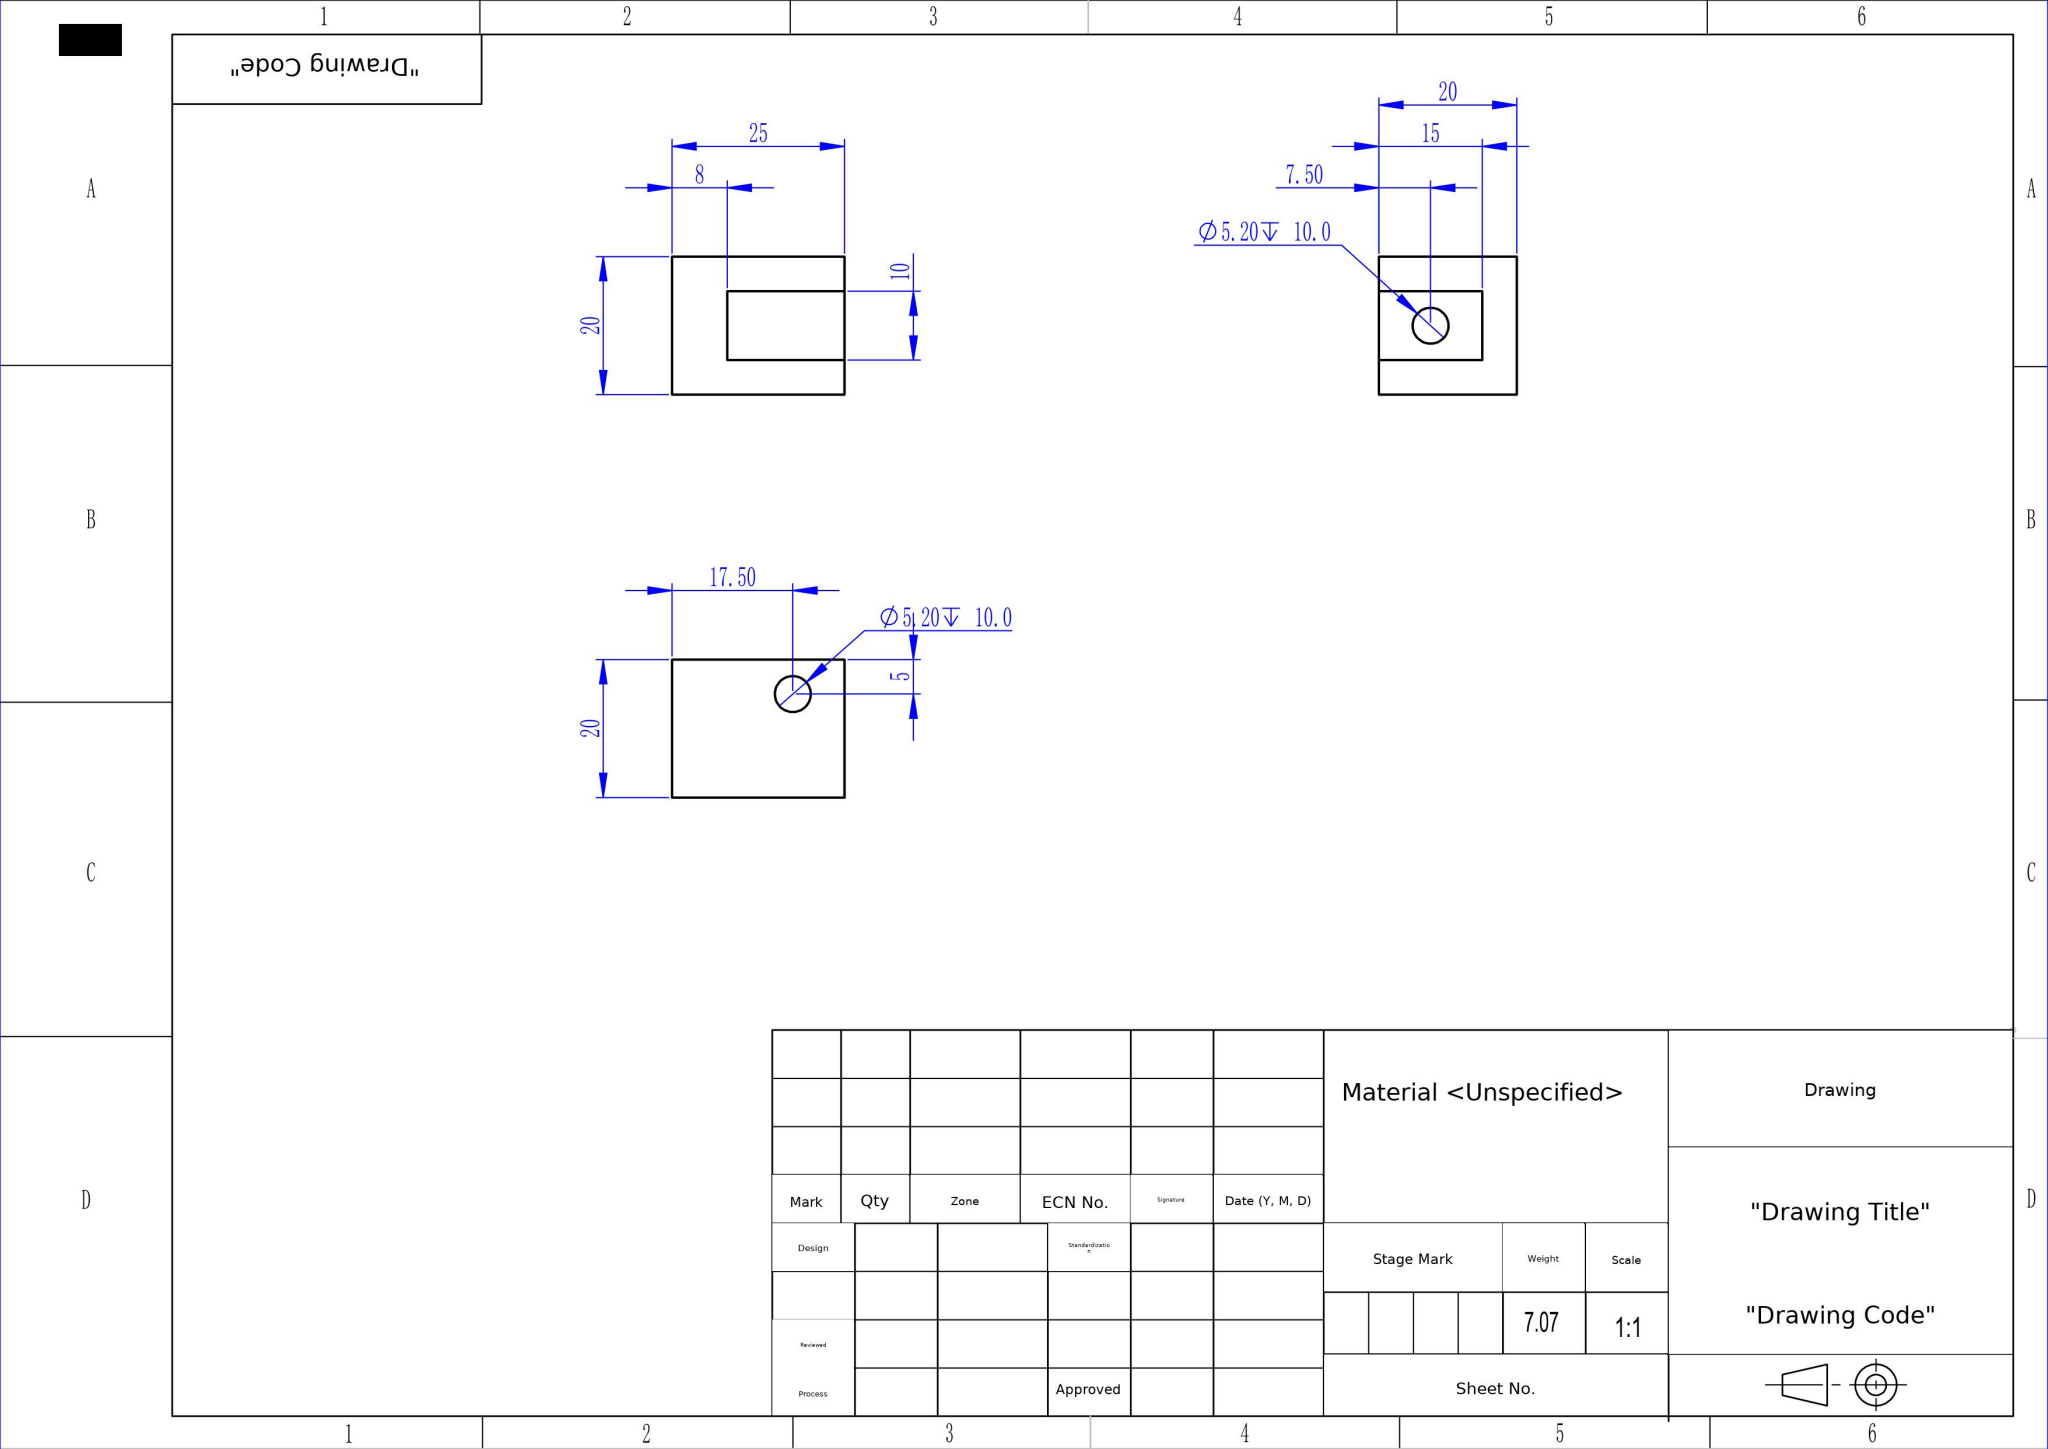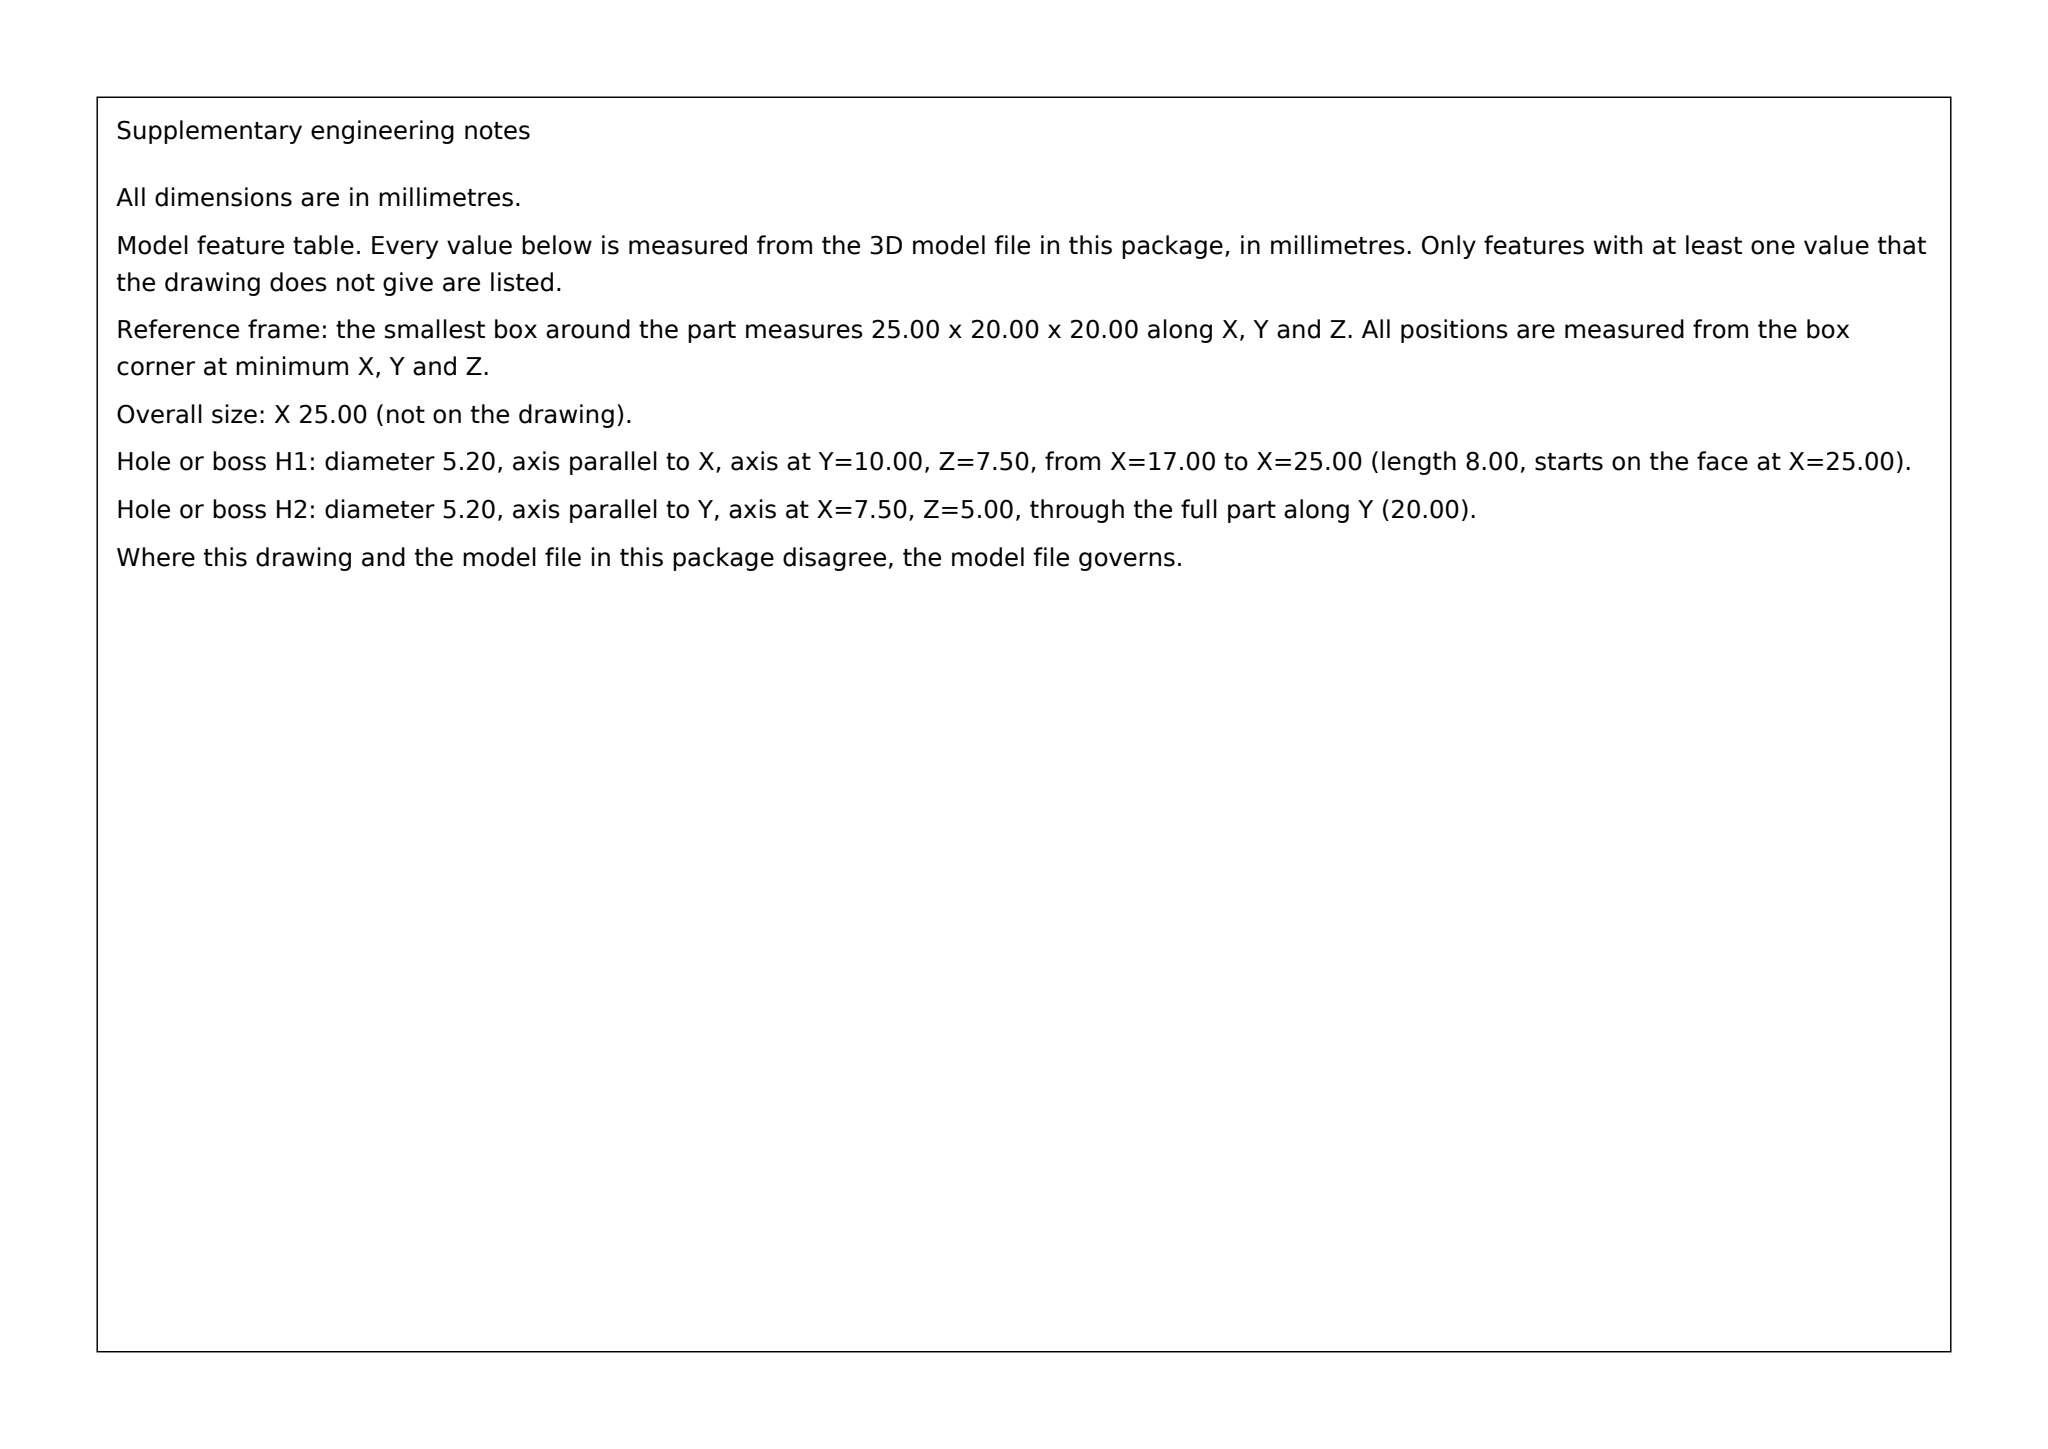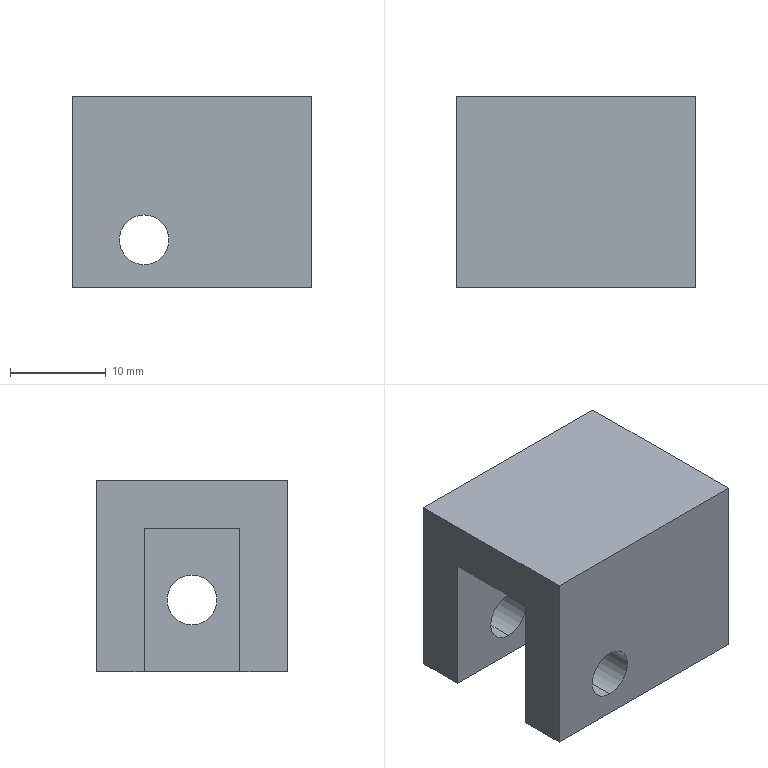Part | SolidWorks | mm | 1 solid | 16 faces | box 25 x 20 x 20 mm | volume 7068 mm3 | plane 10 | cylinder 6 | commonest cylinder face diameters 5.2 x6
build123d program:
from build123d import *

# Parameters (mm, degrees)
SKETCH1_W               = 20
SKETCH1_H               = 20
BOSS_EXTRUDE1_DEPTH     = 25
SKETCH2_W               = 17
SKETCH2_H               = 5
CUT_EXTRUDE1_DEPTH      = 15
SKETCH3_R               = 2.6
CUT_EXTRUDE2_DEPTH      = 10
CUT_EXTRUDE3_DEPTH      = 15
CUT_EXTRUDE3_DEPTH_BACK = 10
SKETCH5_R               = 2.6


with BuildPart() as part:
    # Sketch1 → Boss-Extrude1 (new body)
    with BuildSketch(Plane(origin=(0, 0, 0), x_dir=(0, 0, -1), z_dir=(1, 0, 0))):
        Rectangle(SKETCH1_W, SKETCH1_H)
    extrude(amount=BOSS_EXTRUDE1_DEPTH)

    # Sketch2 → Cut-Extrude1 (cut)
    with BuildSketch(Plane(origin=(0, 0, -10), x_dir=(-1, 0, 0), z_dir=(0, 0, -1))):
        with Locations((-8.5, 2.5)):
            Rectangle(SKETCH2_W, SKETCH2_H)
        with Locations((-8.5, -2.5)):
            Rectangle(SKETCH2_W, SKETCH2_H)
    extrude(amount=-CUT_EXTRUDE1_DEPTH, mode=Mode.SUBTRACT)

    # Sketch3 → Cut-Extrude2 (cut)
    with BuildSketch(Plane.ZY.offset(-17)):
        with Locations((-2.5, 0)):
            Circle(SKETCH3_R)
    extrude(amount=-CUT_EXTRUDE2_DEPTH, mode=Mode.SUBTRACT)

    # Sketch5 → Cut-Extrude3 (cut, two sides: drawn at the far end of the back side and taken through both)
    with BuildSketch(Plane(origin=(0, -5, 0), x_dir=(1, 0, 0), z_dir=(0, 1, 0)).offset(-CUT_EXTRUDE3_DEPTH_BACK)):
        with Locations(Location((7.5, 5, 0), (0, 0, 270))):
            Circle(SKETCH5_R)
    extrude(amount=CUT_EXTRUDE3_DEPTH + CUT_EXTRUDE3_DEPTH_BACK, mode=Mode.SUBTRACT)


solid = part.part
STEP:
#1=CARTESIAN_POINT('',(7.5,10.,-7.6));
#2=VERTEX_POINT('',#1);
#3=CARTESIAN_POINT('',(7.5,10.,-2.4));
#4=VERTEX_POINT('',#3);
#5=CARTESIAN_POINT('',(7.5,10.,-5.));
#6=DIRECTION('',(0.,1.,0.));
#7=DIRECTION('',(0.,0.,1.));
#8=AXIS2_PLACEMENT_3D('',#5,#6,#7);
#9=CIRCLE('',#8,2.6);
#10=EDGE_CURVE('',#2,#4,#9,.T.);
#11=ORIENTED_EDGE('',*,*,#10,.T.);
#12=CARTESIAN_POINT('',(7.5,5.,-2.4));
#13=VERTEX_POINT('',#12);
#14=CARTESIAN_POINT('',(7.5,10.,-2.4));
#15=DIRECTION('',(0.,-1.,-0.));
#16=VECTOR('',#15,1000.);
#17=LINE('',#14,#16);
#18=EDGE_CURVE('',#4,#13,#17,.T.);
#19=ORIENTED_EDGE('',*,*,#18,.T.);
#20=CARTESIAN_POINT('',(7.5,5.,-7.6));
#21=VERTEX_POINT('',#20);
#22=CARTESIAN_POINT('',(7.5,5.,-5.));
#23=DIRECTION('',(-0.,-1.,-0.));
#24=DIRECTION('',(0.,-0.,1.));
#25=AXIS2_PLACEMENT_3D('',#22,#23,#24);
#26=CIRCLE('',#25,2.6);
#27=EDGE_CURVE('',#13,#21,#26,.T.);
#28=ORIENTED_EDGE('',*,*,#27,.T.);
#29=CARTESIAN_POINT('',(7.5,10.,-7.6));
#30=DIRECTION('',(0.,-1.,-0.));
#31=VECTOR('',#30,1000.);
#32=LINE('',#29,#31);
#33=EDGE_CURVE('',#2,#21,#32,.T.);
#34=ORIENTED_EDGE('',*,*,#33,.F.);
#35=EDGE_LOOP('',(#11,#19,#28,#34));
#36=FACE_OUTER_BOUND('',#35,.T.);
#37=CARTESIAN_POINT('',(7.5,10.,-5.));
#38=DIRECTION('',(0.,-1.,-0.));
#39=DIRECTION('',(0.,0.,-1.));
#40=AXIS2_PLACEMENT_3D('',#37,#38,#39);
#41=CYLINDRICAL_SURFACE('',#40,2.6);
#42=ADVANCED_FACE('',(#36),#41,.F.);
#43=CARTESIAN_POINT('',(7.5,-5.,-2.4));
#44=VERTEX_POINT('',#43);
#45=CARTESIAN_POINT('',(7.5,-5.,-7.6));
#46=VERTEX_POINT('',#45);
#47=CARTESIAN_POINT('',(7.5,-5.,-5.));
#48=DIRECTION('',(-0.,-1.,-0.));
#49=DIRECTION('',(0.,-0.,1.));
#50=AXIS2_PLACEMENT_3D('',#47,#48,#49);
#51=CIRCLE('',#50,2.6);
#52=EDGE_CURVE('',#44,#46,#51,.T.);
#53=ORIENTED_EDGE('',*,*,#52,.F.);
#54=CARTESIAN_POINT('',(7.5,-10.,-2.4));
#55=VERTEX_POINT('',#54);
#56=CARTESIAN_POINT('',(7.5,10.,-2.4));
#57=DIRECTION('',(0.,-1.,-0.));
#58=VECTOR('',#57,1000.);
#59=LINE('',#56,#58);
#60=EDGE_CURVE('',#44,#55,#59,.T.);
#61=ORIENTED_EDGE('',*,*,#60,.T.);
#62=CARTESIAN_POINT('',(7.5,-10.,-7.6));
#63=VERTEX_POINT('',#62);
#64=CARTESIAN_POINT('',(7.5,-10.,-5.));
#65=DIRECTION('',(0.,-1.,0.));
#66=DIRECTION('',(0.,0.,1.));
#67=AXIS2_PLACEMENT_3D('',#64,#65,#66);
#68=CIRCLE('',#67,2.6);
#69=EDGE_CURVE('',#55,#63,#68,.T.);
#70=ORIENTED_EDGE('',*,*,#69,.T.);
#71=CARTESIAN_POINT('',(7.5,10.,-7.6));
#72=DIRECTION('',(0.,-1.,-0.));
#73=VECTOR('',#72,1000.);
#74=LINE('',#71,#73);
#75=EDGE_CURVE('',#46,#63,#74,.T.);
#76=ORIENTED_EDGE('',*,*,#75,.F.);
#77=EDGE_LOOP('',(#53,#61,#70,#76));
#78=FACE_OUTER_BOUND('',#77,.T.);
#79=CARTESIAN_POINT('',(7.5,10.,-5.));
#80=DIRECTION('',(0.,-1.,-0.));
#81=DIRECTION('',(0.,0.,-1.));
#82=AXIS2_PLACEMENT_3D('',#79,#80,#81);
#83=CYLINDRICAL_SURFACE('',#82,2.6);
#84=ADVANCED_FACE('',(#78),#83,.F.);
#85=CARTESIAN_POINT('',(25.,0.,0.1));
#86=VERTEX_POINT('',#85);
#87=CARTESIAN_POINT('',(25.,0.,-5.1));
#88=VERTEX_POINT('',#87);
#89=CARTESIAN_POINT('',(25.,0.,-2.5));
#90=DIRECTION('',(1.,0.,0.));
#91=DIRECTION('',(0.,0.,-1.));
#92=AXIS2_PLACEMENT_3D('',#89,#90,#91);
#93=CIRCLE('',#92,2.6);
#94=EDGE_CURVE('',#86,#88,#93,.T.);
#95=ORIENTED_EDGE('',*,*,#94,.T.);
#96=CARTESIAN_POINT('',(17.,0.,-5.1));
#97=VERTEX_POINT('',#96);
#98=CARTESIAN_POINT('',(27.,0.,-5.1));
#99=DIRECTION('',(-1.,0.,0.));
#100=VECTOR('',#99,1000.);
#101=LINE('',#98,#100);
#102=EDGE_CURVE('',#88,#97,#101,.T.);
#103=ORIENTED_EDGE('',*,*,#102,.T.);
#104=CARTESIAN_POINT('',(17.,0.,0.1));
#105=VERTEX_POINT('',#104);
#106=CARTESIAN_POINT('',(17.,0.,-2.5));
#107=DIRECTION('',(-1.,0.,0.));
#108=DIRECTION('',(0.,0.,1.));
#109=AXIS2_PLACEMENT_3D('',#106,#107,#108);
#110=CIRCLE('',#109,2.6);
#111=EDGE_CURVE('',#97,#105,#110,.T.);
#112=ORIENTED_EDGE('',*,*,#111,.T.);
#113=CARTESIAN_POINT('',(27.,0.,0.1));
#114=DIRECTION('',(-1.,0.,0.));
#115=VECTOR('',#114,1000.);
#116=LINE('',#113,#115);
#117=EDGE_CURVE('',#86,#105,#116,.T.);
#118=ORIENTED_EDGE('',*,*,#117,.F.);
#119=EDGE_LOOP('',(#95,#103,#112,#118));
#120=FACE_OUTER_BOUND('',#119,.T.);
#121=CARTESIAN_POINT('',(27.,0.,-2.5));
#122=DIRECTION('',(-1.,0.,0.));
#123=DIRECTION('',(0.,0.,1.));
#124=AXIS2_PLACEMENT_3D('',#121,#122,#123);
#125=CYLINDRICAL_SURFACE('',#124,2.6);
#126=ADVANCED_FACE('',(#120),#125,.F.);
#127=CARTESIAN_POINT('',(17.,-5.,-10.));
#128=VERTEX_POINT('',#127);
#129=CARTESIAN_POINT('',(17.,5.,-10.));
#130=VERTEX_POINT('',#129);
#131=CARTESIAN_POINT('',(17.,0.,-10.));
#132=DIRECTION('',(0.,1.,0.));
#133=VECTOR('',#132,1000.);
#134=LINE('',#131,#133);
#135=EDGE_CURVE('',#128,#130,#134,.T.);
#136=ORIENTED_EDGE('',*,*,#135,.T.);
#137=CARTESIAN_POINT('',(0.,5.,-10.));
#138=VERTEX_POINT('',#137);
#139=CARTESIAN_POINT('',(0.,5.,-10.));
#140=DIRECTION('',(1.,-0.,-0.));
#141=VECTOR('',#140,1000.);
#142=LINE('',#139,#141);
#143=EDGE_CURVE('',#138,#130,#142,.T.);
#144=ORIENTED_EDGE('',*,*,#143,.F.);
#145=CARTESIAN_POINT('',(0.,10.,-10.));
#146=VERTEX_POINT('',#145);
#147=CARTESIAN_POINT('',(0.,10.,-10.));
#148=DIRECTION('',(0.,1.,0.));
#149=VECTOR('',#148,1000.);
#150=LINE('',#147,#149);
#151=EDGE_CURVE('',#138,#146,#150,.T.);
#152=ORIENTED_EDGE('',*,*,#151,.T.);
#153=CARTESIAN_POINT('',(25.,10.,-10.));
#154=VERTEX_POINT('',#153);
#155=CARTESIAN_POINT('',(25.,10.,-10.));
#156=DIRECTION('',(-1.,0.,0.));
#157=VECTOR('',#156,1000.);
#158=LINE('',#155,#157);
#159=EDGE_CURVE('',#154,#146,#158,.T.);
#160=ORIENTED_EDGE('',*,*,#159,.F.);
#161=CARTESIAN_POINT('',(25.,-10.,-10.));
#162=VERTEX_POINT('',#161);
#163=CARTESIAN_POINT('',(25.,10.,-10.));
#164=DIRECTION('',(0.,1.,0.));
#165=VECTOR('',#164,1000.);
#166=LINE('',#163,#165);
#167=EDGE_CURVE('',#162,#154,#166,.T.);
#168=ORIENTED_EDGE('',*,*,#167,.F.);
#169=CARTESIAN_POINT('',(0.,-10.,-10.));
#170=VERTEX_POINT('',#169);
#171=CARTESIAN_POINT('',(25.,-10.,-10.));
#172=DIRECTION('',(-1.,0.,0.));
#173=VECTOR('',#172,1000.);
#174=LINE('',#171,#173);
#175=EDGE_CURVE('',#162,#170,#174,.T.);
#176=ORIENTED_EDGE('',*,*,#175,.T.);
#177=CARTESIAN_POINT('',(0.,-5.,-10.));
#178=VERTEX_POINT('',#177);
#179=CARTESIAN_POINT('',(0.,10.,-10.));
#180=DIRECTION('',(0.,1.,0.));
#181=VECTOR('',#180,1000.);
#182=LINE('',#179,#181);
#183=EDGE_CURVE('',#170,#178,#182,.T.);
#184=ORIENTED_EDGE('',*,*,#183,.T.);
#185=CARTESIAN_POINT('',(-0.,-5.,-10.));
#186=DIRECTION('',(1.,-0.,0.));
#187=VECTOR('',#186,1000.);
#188=LINE('',#185,#187);
#189=EDGE_CURVE('',#178,#128,#188,.T.);
#190=ORIENTED_EDGE('',*,*,#189,.T.);
#191=EDGE_LOOP('',(#136,#144,#152,#160,#168,#176,#184,#190));
#192=FACE_OUTER_BOUND('',#191,.T.);
#193=CARTESIAN_POINT('',(25.,10.,-10.));
#194=DIRECTION('',(0.,-0.,1.));
#195=DIRECTION('',(0.,-1.,-0.));
#196=AXIS2_PLACEMENT_3D('',#193,#194,#195);
#197=PLANE('',#196);
#198=ADVANCED_FACE('',(#192),#197,.F.);
#199=ORIENTED_EDGE('',*,*,#10,.F.);
#200=CARTESIAN_POINT('',(7.5,10.,-5.));
#201=DIRECTION('',(0.,1.,0.));
#202=DIRECTION('',(0.,0.,1.));
#203=AXIS2_PLACEMENT_3D('',#200,#201,#202);
#204=CIRCLE('',#203,2.6);
#205=EDGE_CURVE('',#4,#2,#204,.T.);
#206=ORIENTED_EDGE('',*,*,#205,.F.);
#207=EDGE_LOOP('',(#199,#206));
#208=FACE_BOUND('',#207,.T.);
#209=CARTESIAN_POINT('',(0.,10.,10.));
#210=VERTEX_POINT('',#209);
#211=CARTESIAN_POINT('',(0.,10.,10.));
#212=DIRECTION('',(0.,0.,1.));
#213=VECTOR('',#212,1000.);
#214=LINE('',#211,#213);
#215=EDGE_CURVE('',#146,#210,#214,.T.);
#216=ORIENTED_EDGE('',*,*,#215,.T.);
#217=CARTESIAN_POINT('',(25.,10.,10.));
#218=VERTEX_POINT('',#217);
#219=CARTESIAN_POINT('',(25.,10.,10.));
#220=DIRECTION('',(-1.,0.,0.));
#221=VECTOR('',#220,1000.);
#222=LINE('',#219,#221);
#223=EDGE_CURVE('',#218,#210,#222,.T.);
#224=ORIENTED_EDGE('',*,*,#223,.F.);
#225=CARTESIAN_POINT('',(25.,10.,10.));
#226=DIRECTION('',(0.,0.,1.));
#227=VECTOR('',#226,1000.);
#228=LINE('',#225,#227);
#229=EDGE_CURVE('',#154,#218,#228,.T.);
#230=ORIENTED_EDGE('',*,*,#229,.F.);
#231=ORIENTED_EDGE('',*,*,#159,.T.);
#232=EDGE_LOOP('',(#216,#224,#230,#231));
#233=FACE_OUTER_BOUND('',#232,.T.);
#234=CARTESIAN_POINT('',(25.,10.,10.));
#235=DIRECTION('',(0.,-1.,0.));
#236=DIRECTION('',(0.,0.,-1.));
#237=AXIS2_PLACEMENT_3D('',#234,#235,#236);
#238=PLANE('',#237);
#239=ADVANCED_FACE('',(#208,#233),#238,.F.);
#240=CARTESIAN_POINT('',(0.,-10.,10.));
#241=VERTEX_POINT('',#240);
#242=CARTESIAN_POINT('',(0.,10.,10.));
#243=DIRECTION('',(0.,-1.,-0.));
#244=VECTOR('',#243,1000.);
#245=LINE('',#242,#244);
#246=EDGE_CURVE('',#210,#241,#245,.T.);
#247=ORIENTED_EDGE('',*,*,#246,.T.);
#248=CARTESIAN_POINT('',(25.,-10.,10.));
#249=VERTEX_POINT('',#248);
#250=CARTESIAN_POINT('',(25.,-10.,10.));
#251=DIRECTION('',(-1.,0.,0.));
#252=VECTOR('',#251,1000.);
#253=LINE('',#250,#252);
#254=EDGE_CURVE('',#249,#241,#253,.T.);
#255=ORIENTED_EDGE('',*,*,#254,.F.);
#256=CARTESIAN_POINT('',(25.,10.,10.));
#257=DIRECTION('',(0.,-1.,-0.));
#258=VECTOR('',#257,1000.);
#259=LINE('',#256,#258);
#260=EDGE_CURVE('',#218,#249,#259,.T.);
#261=ORIENTED_EDGE('',*,*,#260,.F.);
#262=ORIENTED_EDGE('',*,*,#223,.T.);
#263=EDGE_LOOP('',(#247,#255,#261,#262));
#264=FACE_OUTER_BOUND('',#263,.T.);
#265=CARTESIAN_POINT('',(25.,10.,10.));
#266=DIRECTION('',(0.,0.,-1.));
#267=DIRECTION('',(0.,1.,0.));
#268=AXIS2_PLACEMENT_3D('',#265,#266,#267);
#269=PLANE('',#268);
#270=ADVANCED_FACE('',(#264),#269,.F.);
#271=CARTESIAN_POINT('',(7.5,-10.,-5.));
#272=DIRECTION('',(0.,-1.,0.));
#273=DIRECTION('',(0.,0.,1.));
#274=AXIS2_PLACEMENT_3D('',#271,#272,#273);
#275=CIRCLE('',#274,2.6);
#276=EDGE_CURVE('',#63,#55,#275,.T.);
#277=ORIENTED_EDGE('',*,*,#276,.F.);
#278=ORIENTED_EDGE('',*,*,#69,.F.);
#279=EDGE_LOOP('',(#277,#278));
#280=FACE_BOUND('',#279,.T.);
#281=CARTESIAN_POINT('',(0.,-10.,10.));
#282=DIRECTION('',(0.,0.,-1.));
#283=VECTOR('',#282,1000.);
#284=LINE('',#281,#283);
#285=EDGE_CURVE('',#241,#170,#284,.T.);
#286=ORIENTED_EDGE('',*,*,#285,.T.);
#287=ORIENTED_EDGE('',*,*,#175,.F.);
#288=CARTESIAN_POINT('',(25.,-10.,10.));
#289=DIRECTION('',(0.,0.,-1.));
#290=VECTOR('',#289,1000.);
#291=LINE('',#288,#290);
#292=EDGE_CURVE('',#249,#162,#291,.T.);
#293=ORIENTED_EDGE('',*,*,#292,.F.);
#294=ORIENTED_EDGE('',*,*,#254,.T.);
#295=EDGE_LOOP('',(#286,#287,#293,#294));
#296=FACE_OUTER_BOUND('',#295,.T.);
#297=CARTESIAN_POINT('',(25.,-10.,10.));
#298=DIRECTION('',(0.,1.,0.));
#299=DIRECTION('',(0.,0.,1.));
#300=AXIS2_PLACEMENT_3D('',#297,#298,#299);
#301=PLANE('',#300);
#302=ADVANCED_FACE('',(#280,#296),#301,.F.);
#303=ORIENTED_EDGE('',*,*,#94,.F.);
#304=CARTESIAN_POINT('',(25.,0.,-2.5));
#305=DIRECTION('',(1.,0.,0.));
#306=DIRECTION('',(0.,0.,-1.));
#307=AXIS2_PLACEMENT_3D('',#304,#305,#306);
#308=CIRCLE('',#307,2.6);
#309=EDGE_CURVE('',#88,#86,#308,.T.);
#310=ORIENTED_EDGE('',*,*,#309,.F.);
#311=EDGE_LOOP('',(#303,#310));
#312=FACE_BOUND('',#311,.T.);
#313=ORIENTED_EDGE('',*,*,#167,.T.);
#314=ORIENTED_EDGE('',*,*,#229,.T.);
#315=ORIENTED_EDGE('',*,*,#260,.T.);
#316=ORIENTED_EDGE('',*,*,#292,.T.);
#317=EDGE_LOOP('',(#313,#314,#315,#316));
#318=FACE_OUTER_BOUND('',#317,.T.);
#319=CARTESIAN_POINT('',(25.,0.,0.));
#320=DIRECTION('',(1.,0.,0.));
#321=DIRECTION('',(0.,0.,-1.));
#322=AXIS2_PLACEMENT_3D('',#319,#320,#321);
#323=PLANE('',#322);
#324=ADVANCED_FACE('',(#312,#318),#323,.T.);
#325=ORIENTED_EDGE('',*,*,#151,.F.);
#326=CARTESIAN_POINT('',(0.,5.,5.));
#327=VERTEX_POINT('',#326);
#328=CARTESIAN_POINT('',(0.,5.,5.));
#329=DIRECTION('',(0.,0.,-1.));
#330=VECTOR('',#329,1000.);
#331=LINE('',#328,#330);
#332=EDGE_CURVE('',#327,#138,#331,.T.);
#333=ORIENTED_EDGE('',*,*,#332,.F.);
#334=CARTESIAN_POINT('',(0.,-5.,5.));
#335=VERTEX_POINT('',#334);
#336=CARTESIAN_POINT('',(0.,-0.,5.));
#337=DIRECTION('',(0.,1.,0.));
#338=VECTOR('',#337,1000.);
#339=LINE('',#336,#338);
#340=EDGE_CURVE('',#335,#327,#339,.T.);
#341=ORIENTED_EDGE('',*,*,#340,.F.);
#342=CARTESIAN_POINT('',(0.,-5.,5.));
#343=DIRECTION('',(0.,0.,-1.));
#344=VECTOR('',#343,1000.);
#345=LINE('',#342,#344);
#346=EDGE_CURVE('',#335,#178,#345,.T.);
#347=ORIENTED_EDGE('',*,*,#346,.T.);
#348=ORIENTED_EDGE('',*,*,#183,.F.);
#349=ORIENTED_EDGE('',*,*,#285,.F.);
#350=ORIENTED_EDGE('',*,*,#246,.F.);
#351=ORIENTED_EDGE('',*,*,#215,.F.);
#352=EDGE_LOOP('',(#325,#333,#341,#347,#348,#349,#350,#351));
#353=FACE_OUTER_BOUND('',#352,.T.);
#354=CARTESIAN_POINT('',(0.,0.,0.));
#355=DIRECTION('',(1.,0.,0.));
#356=DIRECTION('',(0.,0.,-1.));
#357=AXIS2_PLACEMENT_3D('',#354,#355,#356);
#358=PLANE('',#357);
#359=ADVANCED_FACE('',(#353),#358,.F.);
#360=CARTESIAN_POINT('',(17.,0.,-2.5));
#361=DIRECTION('',(-1.,0.,0.));
#362=DIRECTION('',(0.,0.,1.));
#363=AXIS2_PLACEMENT_3D('',#360,#361,#362);
#364=CIRCLE('',#363,2.6);
#365=EDGE_CURVE('',#105,#97,#364,.T.);
#366=ORIENTED_EDGE('',*,*,#365,.F.);
#367=ORIENTED_EDGE('',*,*,#111,.F.);
#368=EDGE_LOOP('',(#366,#367));
#369=FACE_BOUND('',#368,.T.);
#370=ORIENTED_EDGE('',*,*,#135,.F.);
#371=CARTESIAN_POINT('',(17.,-5.,5.));
#372=VERTEX_POINT('',#371);
#373=CARTESIAN_POINT('',(17.,-5.,5.));
#374=DIRECTION('',(0.,0.,-1.));
#375=VECTOR('',#374,1000.);
#376=LINE('',#373,#375);
#377=EDGE_CURVE('',#372,#128,#376,.T.);
#378=ORIENTED_EDGE('',*,*,#377,.F.);
#379=CARTESIAN_POINT('',(17.,5.,5.));
#380=VERTEX_POINT('',#379);
#381=CARTESIAN_POINT('',(17.,-0.,5.));
#382=DIRECTION('',(0.,1.,0.));
#383=VECTOR('',#382,1000.);
#384=LINE('',#381,#383);
#385=EDGE_CURVE('',#372,#380,#384,.T.);
#386=ORIENTED_EDGE('',*,*,#385,.T.);
#387=CARTESIAN_POINT('',(17.,5.,5.));
#388=DIRECTION('',(0.,0.,-1.));
#389=VECTOR('',#388,1000.);
#390=LINE('',#387,#389);
#391=EDGE_CURVE('',#380,#130,#390,.T.);
#392=ORIENTED_EDGE('',*,*,#391,.T.);
#393=EDGE_LOOP('',(#370,#378,#386,#392));
#394=FACE_OUTER_BOUND('',#393,.T.);
#395=CARTESIAN_POINT('',(17.,-0.,5.));
#396=DIRECTION('',(-1.,0.,0.));
#397=DIRECTION('',(0.,0.,1.));
#398=AXIS2_PLACEMENT_3D('',#395,#396,#397);
#399=PLANE('',#398);
#400=ADVANCED_FACE('',(#369,#394),#399,.T.);
#401=CARTESIAN_POINT('',(7.5,5.,-5.));
#402=DIRECTION('',(-0.,-1.,-0.));
#403=DIRECTION('',(0.,-0.,1.));
#404=AXIS2_PLACEMENT_3D('',#401,#402,#403);
#405=CIRCLE('',#404,2.6);
#406=EDGE_CURVE('',#21,#13,#405,.T.);
#407=ORIENTED_EDGE('',*,*,#406,.F.);
#408=ORIENTED_EDGE('',*,*,#27,.F.);
#409=EDGE_LOOP('',(#407,#408));
#410=FACE_BOUND('',#409,.T.);
#411=ORIENTED_EDGE('',*,*,#143,.T.);
#412=ORIENTED_EDGE('',*,*,#391,.F.);
#413=CARTESIAN_POINT('',(0.,5.,5.));
#414=DIRECTION('',(1.,-0.,-0.));
#415=VECTOR('',#414,1000.);
#416=LINE('',#413,#415);
#417=EDGE_CURVE('',#327,#380,#416,.T.);
#418=ORIENTED_EDGE('',*,*,#417,.F.);
#419=ORIENTED_EDGE('',*,*,#332,.T.);
#420=EDGE_LOOP('',(#411,#412,#418,#419));
#421=FACE_OUTER_BOUND('',#420,.T.);
#422=CARTESIAN_POINT('',(0.,5.,5.));
#423=DIRECTION('',(0.,1.,0.));
#424=DIRECTION('',(0.,-0.,1.));
#425=AXIS2_PLACEMENT_3D('',#422,#423,#424);
#426=PLANE('',#425);
#427=ADVANCED_FACE('',(#410,#421),#426,.F.);
#428=CARTESIAN_POINT('',(7.5,-5.,-5.));
#429=DIRECTION('',(-0.,-1.,-0.));
#430=DIRECTION('',(0.,-0.,1.));
#431=AXIS2_PLACEMENT_3D('',#428,#429,#430);
#432=CIRCLE('',#431,2.6);
#433=EDGE_CURVE('',#46,#44,#432,.T.);
#434=ORIENTED_EDGE('',*,*,#433,.T.);
#435=ORIENTED_EDGE('',*,*,#52,.T.);
#436=EDGE_LOOP('',(#434,#435));
#437=FACE_BOUND('',#436,.T.);
#438=ORIENTED_EDGE('',*,*,#189,.F.);
#439=ORIENTED_EDGE('',*,*,#346,.F.);
#440=CARTESIAN_POINT('',(-0.,-5.,5.));
#441=DIRECTION('',(1.,-0.,0.));
#442=VECTOR('',#441,1000.);
#443=LINE('',#440,#442);
#444=EDGE_CURVE('',#335,#372,#443,.T.);
#445=ORIENTED_EDGE('',*,*,#444,.T.);
#446=ORIENTED_EDGE('',*,*,#377,.T.);
#447=EDGE_LOOP('',(#438,#439,#445,#446));
#448=FACE_OUTER_BOUND('',#447,.T.);
#449=CARTESIAN_POINT('',(-0.,-5.,5.));
#450=DIRECTION('',(0.,1.,0.));
#451=DIRECTION('',(0.,-0.,1.));
#452=AXIS2_PLACEMENT_3D('',#449,#450,#451);
#453=PLANE('',#452);
#454=ADVANCED_FACE('',(#437,#448),#453,.T.);
#455=ORIENTED_EDGE('',*,*,#385,.F.);
#456=ORIENTED_EDGE('',*,*,#444,.F.);
#457=ORIENTED_EDGE('',*,*,#340,.T.);
#458=ORIENTED_EDGE('',*,*,#417,.T.);
#459=EDGE_LOOP('',(#455,#456,#457,#458));
#460=FACE_OUTER_BOUND('',#459,.T.);
#461=CARTESIAN_POINT('',(0.,-0.,5.));
#462=DIRECTION('',(0.,0.,-1.));
#463=DIRECTION('',(0.,1.,0.));
#464=AXIS2_PLACEMENT_3D('',#461,#462,#463);
#465=PLANE('',#464);
#466=ADVANCED_FACE('',(#460),#465,.T.);
#467=ORIENTED_EDGE('',*,*,#102,.F.);
#468=ORIENTED_EDGE('',*,*,#309,.T.);
#469=ORIENTED_EDGE('',*,*,#117,.T.);
#470=ORIENTED_EDGE('',*,*,#365,.T.);
#471=EDGE_LOOP('',(#467,#468,#469,#470));
#472=FACE_OUTER_BOUND('',#471,.T.);
#473=CARTESIAN_POINT('',(27.,0.,-2.5));
#474=DIRECTION('',(-1.,0.,0.));
#475=DIRECTION('',(0.,0.,1.));
#476=AXIS2_PLACEMENT_3D('',#473,#474,#475);
#477=CYLINDRICAL_SURFACE('',#476,2.6);
#478=ADVANCED_FACE('',(#472),#477,.F.);
#479=ORIENTED_EDGE('',*,*,#60,.F.);
#480=ORIENTED_EDGE('',*,*,#433,.F.);
#481=ORIENTED_EDGE('',*,*,#75,.T.);
#482=ORIENTED_EDGE('',*,*,#276,.T.);
#483=EDGE_LOOP('',(#479,#480,#481,#482));
#484=FACE_OUTER_BOUND('',#483,.T.);
#485=CARTESIAN_POINT('',(7.5,10.,-5.));
#486=DIRECTION('',(0.,-1.,-0.));
#487=DIRECTION('',(0.,0.,-1.));
#488=AXIS2_PLACEMENT_3D('',#485,#486,#487);
#489=CYLINDRICAL_SURFACE('',#488,2.6);
#490=ADVANCED_FACE('',(#484),#489,.F.);
#491=ORIENTED_EDGE('',*,*,#18,.F.);
#492=ORIENTED_EDGE('',*,*,#205,.T.);
#493=ORIENTED_EDGE('',*,*,#33,.T.);
#494=ORIENTED_EDGE('',*,*,#406,.T.);
#495=EDGE_LOOP('',(#491,#492,#493,#494));
#496=FACE_OUTER_BOUND('',#495,.T.);
#497=CARTESIAN_POINT('',(7.5,10.,-5.));
#498=DIRECTION('',(0.,-1.,-0.));
#499=DIRECTION('',(0.,0.,-1.));
#500=AXIS2_PLACEMENT_3D('',#497,#498,#499);
#501=CYLINDRICAL_SURFACE('',#500,2.6);
#502=ADVANCED_FACE('',(#496),#501,.F.);
#503=CLOSED_SHELL('',(#42,#84,#126,#198,#239,#270,#302,#324,#359,#400,#427,#454,#466,#478,#490,#502));
#504=MANIFOLD_SOLID_BREP('',#503);
#505=CARTESIAN_POINT('',(0.,0.,0.));
#506=DIRECTION('',(0.,0.,1.));
#507=DIRECTION('',(1.,0.,0.));
#508=AXIS2_PLACEMENT_3D('',#505,#506,#507);
#509=(LENGTH_UNIT()NAMED_UNIT(*)SI_UNIT(.MILLI.,.METRE.));
#510=UNCERTAINTY_MEASURE_WITH_UNIT(LENGTH_MEASURE(0.00001),#509,'','');
#511=(NAMED_UNIT(*)PLANE_ANGLE_UNIT()SI_UNIT($,.RADIAN.));
#512=(NAMED_UNIT(*)SI_UNIT($,.STERADIAN.)SOLID_ANGLE_UNIT());
#513=(GEOMETRIC_REPRESENTATION_CONTEXT(3)GLOBAL_UNCERTAINTY_ASSIGNED_CONTEXT((#510))GLOBAL_UNIT_ASSIGNED_CONTEXT((#509,#511,#512))REPRESENTATION_CONTEXT('',''));
#514=ADVANCED_BREP_SHAPE_REPRESENTATION('',(#504,#508),#513);